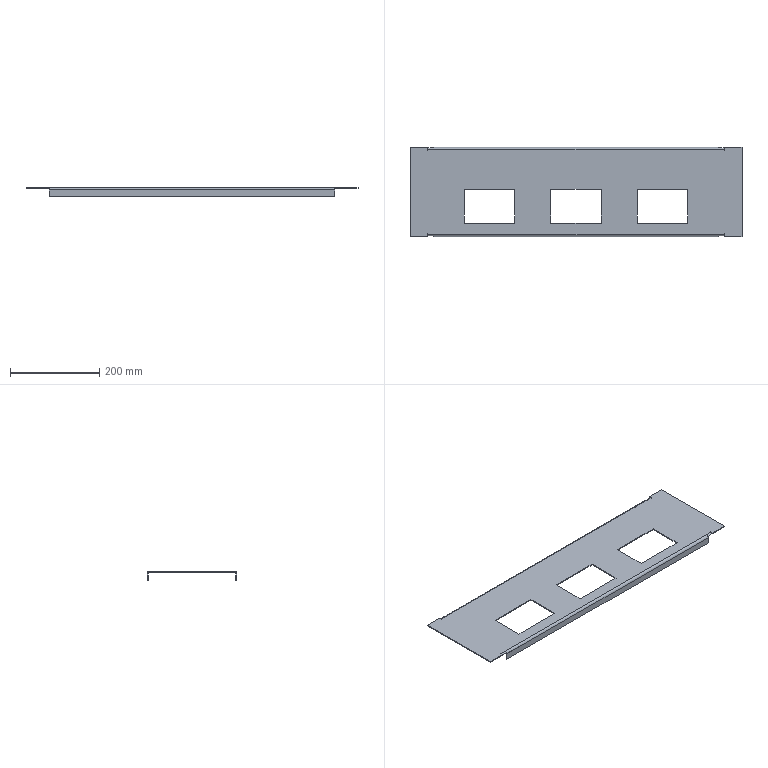Component | SolidWorks | Panel1-2 | 1 solid | 50 faces | volume 286845 mm3 | plane 46 | cylinder 4 | commonest cylinder face diameters 11 x2 7 x2 | material Malleable Cast Iron